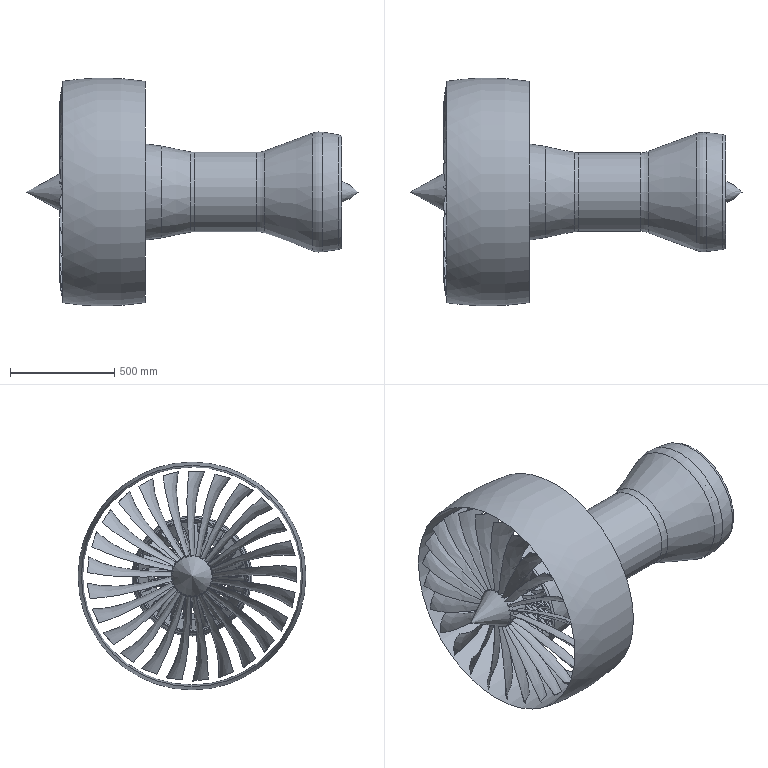Assembly | NX | mm | 5 component files | 5 solids | 928 faces | box 1590.6 x 1092.34 x 1092.34 mm | volume 59886368 mm3 | spline 571 | plane 300 | torus 32 | cylinder 13 | cone 10 | other 2 | commonest cylinder face diameters 60 x4 30 x2 80 x2 200 x2 360 x1 380 x1 130 x1
Bill of materials:
unnamed part 1 | 1 |  | Long slender shaft carrying two groups of bladed rotor discs: five closely spaced bladed stages at one end and two bladed stages at the other end, with an open-ended hollow bore at one end.
unnamed part 2 | 1 |  | Single-stage bladed rotor (fan-like) with a thin disc carrying many slender, twisted, radially swept blades, a pointed conical nose cone on one face, and a hub with a central bore on the other.
unnamed part 3 | 1 |  | Thin shaft connecting two groups of three bladed discs each, with a rounded-to-pointed nose cone at one end and a short cylindrical stub sticking out at the other end.
unnamed part 4 | 1 |  | Thin-walled, open cylindrical ring or band with a large diameter compared with its wall thickness. The outer surface appears to be slightly barrel-curved along its axial length.
unnamed part 5 | 1 |  | Hollow axisymmetric duct with a converging-diverging (waisted) profile: a long gently tapered section at one end, a straight cylindrical throat in the middle, a shorter steeper flared cone, and a short cylindrical lip at the other end.
Mates:
1. fix | Turbofan_Engine 1 component
2. concentric | shaft_with_blades 1 edge | Turbofan_Engine 1 edge
3. angle | shaft_with_blades 1 datumplane | Turbofan_Engine 1 datumplane
4. touch align | comp_and_turb 1 face | shaft_with_blades 1 face
5. distance | comp_and_turb 1 face | shaft_with_blades 1 face
6. touch align | housing 1 face | shaft_with_blades 1 face
7. concentric | main_housing 1 edge | Turbofan_Engine 1 edge
8. angle | main_housing 1 datumplane | housing 1 datumplane